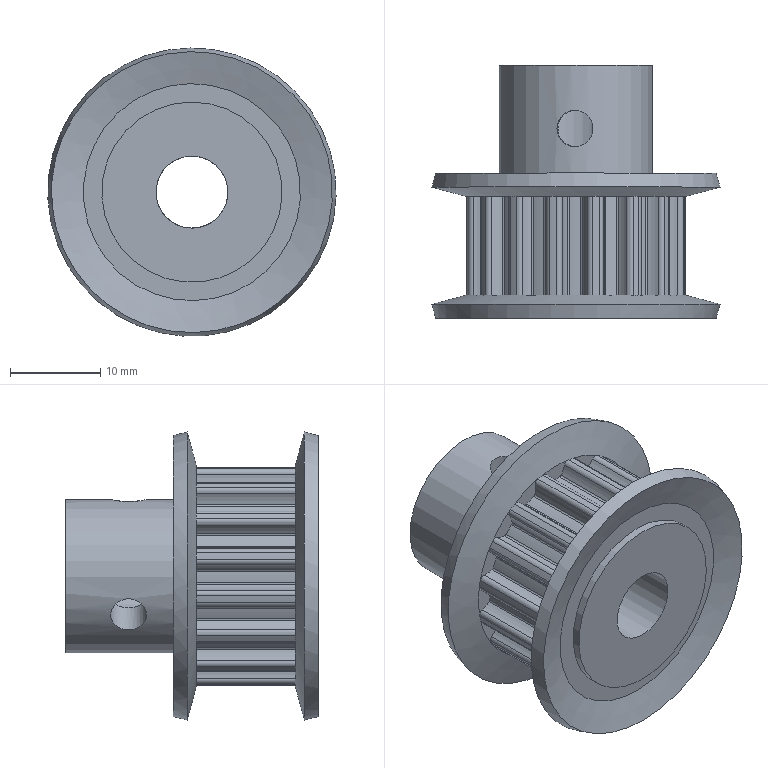Component | NX | SYNCHRONOUS_PULLEY_2 | 1 solid | 177 faces | volume 8720 mm3 | cylinder 134 | plane 37 | cone 6 | commonest cylinder face diameters 1.1 x32 6.55 x32 0.5 x32 24.5 x16 20.96 x16 20 x2 4 x2 17 x1